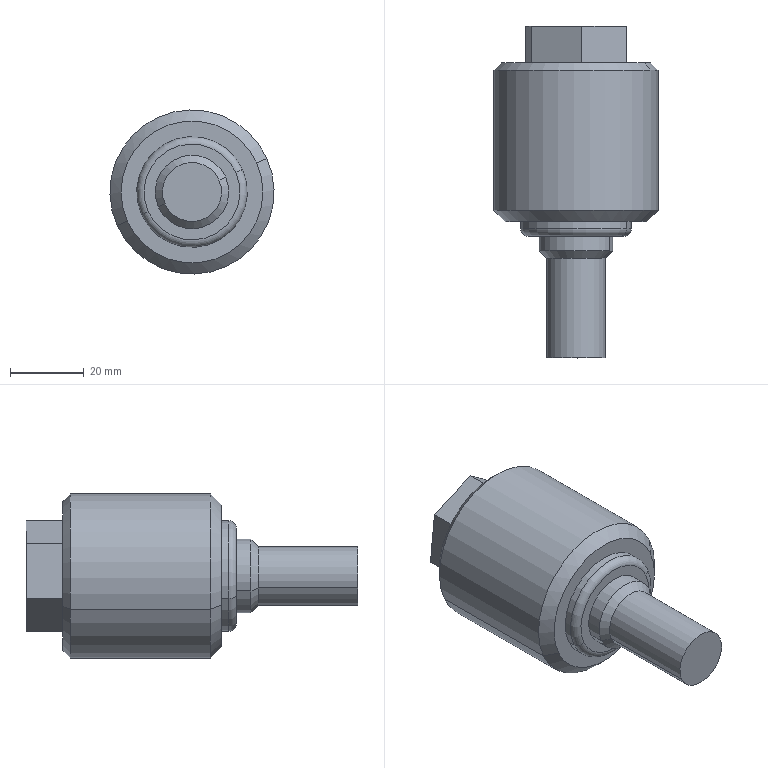Component | SolidWorks | -F-M16150F-1 | 1 solid | 31 faces | box 44.5 x 90 x 44.5 mm | volume 77654 mm3 | plane 11 | cylinder 10 | cone 8 | torus 2 | commonest cylinder face diameters 16 x4 44.5 x2 30 x2 20 x2
STEP:
#1=CARTESIAN_POINT('',(0.8934,52.697,-4.853));
#2=VERTEX_POINT('',#1);
#3=CARTESIAN_POINT('',(1.469,52.697,-4.596));
#4=VERTEX_POINT('',#3);
#5=CARTESIAN_POINT('',(1.181,52.697,-4.724));
#6=DIRECTION('',(-0.,1.,0.));
#7=DIRECTION('',(0.9136,0.,0.4067));
#8=AXIS2_PLACEMENT_3D('',#5,#6,#7);
#9=CIRCLE('',#8,0.315);
#10=EDGE_CURVE('',#2,#4,#9,.T.);
#11=ORIENTED_EDGE('',*,*,#10,.F.);
#12=CARTESIAN_POINT('',(0.8934,53.445,-4.853));
#13=VERTEX_POINT('',#12);
#14=CARTESIAN_POINT('',(0.8934,53.445,-4.853));
#15=DIRECTION('',(-0.,1.,0.));
#16=VECTOR('',#15,39.37);
#17=LINE('',#14,#16);
#18=EDGE_CURVE('',#2,#13,#17,.T.);
#19=ORIENTED_EDGE('',*,*,#18,.T.);
#20=CARTESIAN_POINT('',(1.469,53.445,-4.596));
#21=VERTEX_POINT('',#20);
#22=CARTESIAN_POINT('',(1.181,53.445,-4.724));
#23=DIRECTION('',(-0.,1.,0.));
#24=DIRECTION('',(0.9136,0.,0.4067));
#25=AXIS2_PLACEMENT_3D('',#22,#23,#24);
#26=CIRCLE('',#25,0.315);
#27=EDGE_CURVE('',#13,#21,#26,.T.);
#28=ORIENTED_EDGE('',*,*,#27,.T.);
#29=CARTESIAN_POINT('',(1.469,53.445,-4.596));
#30=DIRECTION('',(-0.,1.,0.));
#31=VECTOR('',#30,39.37);
#32=LINE('',#29,#31);
#33=EDGE_CURVE('',#4,#21,#32,.T.);
#34=ORIENTED_EDGE('',*,*,#33,.F.);
#35=EDGE_LOOP('',(#11,#19,#28,#34));
#36=FACE_OUTER_BOUND('',#35,.T.);
#37=CARTESIAN_POINT('',(1.181,53.445,-4.724));
#38=DIRECTION('',(-0.,1.,0.));
#39=DIRECTION('',(0.9136,0.,0.4067));
#40=AXIS2_PLACEMENT_3D('',#37,#38,#39);
#41=CYLINDRICAL_SURFACE('',#40,0.315);
#42=ADVANCED_FACE('',(#36),#41,.F.);
#43=CARTESIAN_POINT('',(1.181,52.508,-4.724));
#44=VERTEX_POINT('',#43);
#45=CARTESIAN_POINT('',(1.469,52.697,-4.596));
#46=DIRECTION('',(0.7831,0.515,0.3486));
#47=VECTOR('',#46,39.37);
#48=LINE('',#45,#47);
#49=EDGE_CURVE('',#44,#4,#48,.T.);
#50=ORIENTED_EDGE('',*,*,#49,.F.);
#51=CARTESIAN_POINT('',(0.8934,52.697,-4.853));
#52=DIRECTION('',(-0.7831,0.515,-0.3486));
#53=VECTOR('',#52,39.37);
#54=LINE('',#51,#53);
#55=EDGE_CURVE('',#44,#2,#54,.T.);
#56=ORIENTED_EDGE('',*,*,#55,.T.);
#57=ORIENTED_EDGE('',*,*,#10,.T.);
#58=EDGE_LOOP('',(#50,#56,#57));
#59=FACE_OUTER_BOUND('',#58,.T.);
#60=CARTESIAN_POINT('',(1.181,52.697,-4.724));
#61=DIRECTION('',(-0.,1.,0.));
#62=DIRECTION('',(0.9136,0.,0.4067));
#63=AXIS2_PLACEMENT_3D('',#60,#61,#62);
#64=CONICAL_SURFACE('',#63,0.315,1.03);
#65=ADVANCED_FACE('',(#59),#64,.F.);
#66=CARTESIAN_POINT('',(1.909,53.051,-4.4));
#67=VERTEX_POINT('',#66);
#68=CARTESIAN_POINT('',(0.4528,53.051,-5.049));
#69=VERTEX_POINT('',#68);
#70=CARTESIAN_POINT('',(1.181,53.051,-4.724));
#71=DIRECTION('',(-0.,1.,0.));
#72=DIRECTION('',(-0.9136,0.,-0.4067));
#73=AXIS2_PLACEMENT_3D('',#70,#71,#72);
#74=CIRCLE('',#73,0.7972);
#75=EDGE_CURVE('',#67,#69,#74,.T.);
#76=ORIENTED_EDGE('',*,*,#75,.F.);
#77=CARTESIAN_POINT('',(1.981,52.972,-4.368));
#78=VERTEX_POINT('',#77);
#79=CARTESIAN_POINT('',(1.981,52.972,-4.368));
#80=DIRECTION('',(0.646,-0.7071,0.2876));
#81=VECTOR('',#80,39.37);
#82=LINE('',#79,#81);
#83=EDGE_CURVE('',#67,#78,#82,.T.);
#84=ORIENTED_EDGE('',*,*,#83,.T.);
#85=CARTESIAN_POINT('',(0.3808,52.972,-5.081));
#86=VERTEX_POINT('',#85);
#87=CARTESIAN_POINT('',(1.181,52.972,-4.724));
#88=DIRECTION('',(0.,-1.,-0.));
#89=DIRECTION('',(-0.9136,0.,-0.4067));
#90=AXIS2_PLACEMENT_3D('',#87,#88,#89);
#91=CIRCLE('',#90,0.876);
#92=EDGE_CURVE('',#86,#78,#91,.T.);
#93=ORIENTED_EDGE('',*,*,#92,.F.);
#94=CARTESIAN_POINT('',(0.3808,52.972,-5.081));
#95=DIRECTION('',(-0.646,-0.7071,-0.2876));
#96=VECTOR('',#95,39.37);
#97=LINE('',#94,#96);
#98=EDGE_CURVE('',#69,#86,#97,.T.);
#99=ORIENTED_EDGE('',*,*,#98,.F.);
#100=EDGE_LOOP('',(#76,#84,#93,#99));
#101=FACE_OUTER_BOUND('',#100,.T.);
#102=CARTESIAN_POINT('',(1.181,52.972,-4.724));
#103=DIRECTION('',(0.,-1.,-0.));
#104=DIRECTION('',(-0.9136,0.,-0.4067));
#105=AXIS2_PLACEMENT_3D('',#102,#103,#104);
#106=CONICAL_SURFACE('',#105,0.876,0.7854);
#107=ADVANCED_FACE('',(#101),#106,.T.);
#108=CARTESIAN_POINT('',(0.4887,51.358,-5.033));
#109=VERTEX_POINT('',#108);
#110=CARTESIAN_POINT('',(1.873,51.358,-4.416));
#111=VERTEX_POINT('',#110);
#112=CARTESIAN_POINT('',(1.181,51.358,-4.724));
#113=DIRECTION('',(0.,-1.,-0.));
#114=DIRECTION('',(0.9136,0.,0.4067));
#115=AXIS2_PLACEMENT_3D('',#112,#113,#114);
#116=CIRCLE('',#115,0.7579);
#117=EDGE_CURVE('',#109,#111,#116,.T.);
#118=ORIENTED_EDGE('',*,*,#117,.F.);
#119=CARTESIAN_POINT('',(0.3808,51.476,-5.081));
#120=VERTEX_POINT('',#119);
#121=CARTESIAN_POINT('',(0.4887,51.358,-5.033));
#122=DIRECTION('',(-0.646,0.7071,-0.2876));
#123=VECTOR('',#122,39.37);
#124=LINE('',#121,#123);
#125=EDGE_CURVE('',#109,#120,#124,.T.);
#126=ORIENTED_EDGE('',*,*,#125,.T.);
#127=CARTESIAN_POINT('',(1.981,51.476,-4.368));
#128=VERTEX_POINT('',#127);
#129=CARTESIAN_POINT('',(1.181,51.476,-4.724));
#130=DIRECTION('',(-0.,1.,0.));
#131=DIRECTION('',(0.9136,0.,0.4067));
#132=AXIS2_PLACEMENT_3D('',#129,#130,#131);
#133=CIRCLE('',#132,0.876);
#134=EDGE_CURVE('',#128,#120,#133,.T.);
#135=ORIENTED_EDGE('',*,*,#134,.F.);
#136=CARTESIAN_POINT('',(1.873,51.358,-4.416));
#137=DIRECTION('',(0.646,0.7071,0.2876));
#138=VECTOR('',#137,39.37);
#139=LINE('',#136,#138);
#140=EDGE_CURVE('',#111,#128,#139,.T.);
#141=ORIENTED_EDGE('',*,*,#140,.F.);
#142=EDGE_LOOP('',(#118,#126,#135,#141));
#143=FACE_OUTER_BOUND('',#142,.T.);
#144=CARTESIAN_POINT('',(1.181,51.358,-4.724));
#145=DIRECTION('',(-0.,1.,0.));
#146=DIRECTION('',(0.9136,0.,0.4067));
#147=AXIS2_PLACEMENT_3D('',#144,#145,#146);
#148=CONICAL_SURFACE('',#147,0.7579,0.7854);
#149=ADVANCED_FACE('',(#143),#148,.T.);
#150=CARTESIAN_POINT('',(0.7135,51.201,-4.933));
#151=VERTEX_POINT('',#150);
#152=CARTESIAN_POINT('',(1.649,51.201,-4.516));
#153=VERTEX_POINT('',#152);
#154=CARTESIAN_POINT('',(1.181,51.201,-4.724));
#155=DIRECTION('',(0.,-1.,-0.));
#156=DIRECTION('',(0.9136,0.,0.4067));
#157=AXIS2_PLACEMENT_3D('',#154,#155,#156);
#158=CIRCLE('',#157,0.5118);
#159=EDGE_CURVE('',#151,#153,#158,.T.);
#160=ORIENTED_EDGE('',*,*,#159,.F.);
#161=CARTESIAN_POINT('',(0.6416,51.28,-4.965));
#162=VERTEX_POINT('',#161);
#163=CARTESIAN_POINT('',(0.7135,51.28,-4.933));
#164=DIRECTION('',(0.4067,0.,-0.9136));
#165=DIRECTION('',(-0.9136,0.,-0.4067));
#166=AXIS2_PLACEMENT_3D('',#163,#164,#165);
#167=CIRCLE('',#166,0.07874);
#168=EDGE_CURVE('',#151,#162,#167,.T.);
#169=ORIENTED_EDGE('',*,*,#168,.T.);
#170=CARTESIAN_POINT('',(1.721,51.28,-4.484));
#171=VERTEX_POINT('',#170);
#172=CARTESIAN_POINT('',(1.181,51.28,-4.724));
#173=DIRECTION('',(-0.,1.,0.));
#174=DIRECTION('',(0.9136,0.,0.4067));
#175=AXIS2_PLACEMENT_3D('',#172,#173,#174);
#176=CIRCLE('',#175,0.5906);
#177=EDGE_CURVE('',#171,#162,#176,.T.);
#178=ORIENTED_EDGE('',*,*,#177,.F.);
#179=CARTESIAN_POINT('',(1.649,51.28,-4.516));
#180=DIRECTION('',(-0.4067,-0.,0.9136));
#181=DIRECTION('',(0.9136,0.,0.4067));
#182=AXIS2_PLACEMENT_3D('',#179,#180,#181);
#183=CIRCLE('',#182,0.07874);
#184=EDGE_CURVE('',#153,#171,#183,.T.);
#185=ORIENTED_EDGE('',*,*,#184,.F.);
#186=EDGE_LOOP('',(#160,#169,#178,#185));
#187=FACE_OUTER_BOUND('',#186,.T.);
#188=CARTESIAN_POINT('',(1.181,51.28,-4.724));
#189=DIRECTION('',(-0.,1.,0.));
#190=DIRECTION('',(0.9136,-0.,0.4067));
#191=AXIS2_PLACEMENT_3D('',#188,#189,#190);
#192=TOROIDAL_SURFACE('',#191,0.5118,0.07874);
#193=ADVANCED_FACE('',(#187),#192,.T.);
#194=CARTESIAN_POINT('',(0.8934,50.965,-4.853));
#195=VERTEX_POINT('',#194);
#196=CARTESIAN_POINT('',(1.469,50.965,-4.596));
#197=VERTEX_POINT('',#196);
#198=CARTESIAN_POINT('',(1.181,50.965,-4.724));
#199=DIRECTION('',(0.,-1.,-0.));
#200=DIRECTION('',(-0.9136,0.,-0.4067));
#201=AXIS2_PLACEMENT_3D('',#198,#199,#200);
#202=CIRCLE('',#201,0.315);
#203=EDGE_CURVE('',#195,#197,#202,.T.);
#204=ORIENTED_EDGE('',*,*,#203,.F.);
#205=CARTESIAN_POINT('',(0.8214,51.043,-4.885));
#206=VERTEX_POINT('',#205);
#207=CARTESIAN_POINT('',(0.8934,50.965,-4.853));
#208=DIRECTION('',(-0.646,0.7071,-0.2876));
#209=VECTOR('',#208,39.37);
#210=LINE('',#207,#209);
#211=EDGE_CURVE('',#195,#206,#210,.T.);
#212=ORIENTED_EDGE('',*,*,#211,.T.);
#213=CARTESIAN_POINT('',(1.541,51.043,-4.564));
#214=VERTEX_POINT('',#213);
#215=CARTESIAN_POINT('',(1.181,51.043,-4.724));
#216=DIRECTION('',(-0.,1.,0.));
#217=DIRECTION('',(0.9136,0.,0.4067));
#218=AXIS2_PLACEMENT_3D('',#215,#216,#217);
#219=CIRCLE('',#218,0.3937);
#220=EDGE_CURVE('',#214,#206,#219,.T.);
#221=ORIENTED_EDGE('',*,*,#220,.F.);
#222=CARTESIAN_POINT('',(1.469,50.965,-4.596));
#223=DIRECTION('',(0.646,0.7071,0.2876));
#224=VECTOR('',#223,39.37);
#225=LINE('',#222,#224);
#226=EDGE_CURVE('',#197,#214,#225,.T.);
#227=ORIENTED_EDGE('',*,*,#226,.F.);
#228=EDGE_LOOP('',(#204,#212,#221,#227));
#229=FACE_OUTER_BOUND('',#228,.T.);
#230=CARTESIAN_POINT('',(1.181,50.965,-4.724));
#231=DIRECTION('',(-0.,1.,0.));
#232=DIRECTION('',(0.9136,0.,0.4067));
#233=AXIS2_PLACEMENT_3D('',#230,#231,#232);
#234=CONICAL_SURFACE('',#233,0.315,0.7854);
#235=ADVANCED_FACE('',(#229),#234,.T.);
#236=ORIENTED_EDGE('',*,*,#92,.T.);
#237=CARTESIAN_POINT('',(1.981,38.509,-4.368));
#238=DIRECTION('',(0.,-1.,-0.));
#239=VECTOR('',#238,39.37);
#240=LINE('',#237,#239);
#241=EDGE_CURVE('',#78,#128,#240,.T.);
#242=ORIENTED_EDGE('',*,*,#241,.T.);
#243=ORIENTED_EDGE('',*,*,#134,.T.);
#244=CARTESIAN_POINT('',(0.3808,38.509,-5.081));
#245=DIRECTION('',(0.,-1.,-0.));
#246=VECTOR('',#245,39.37);
#247=LINE('',#244,#246);
#248=EDGE_CURVE('',#86,#120,#247,.T.);
#249=ORIENTED_EDGE('',*,*,#248,.F.);
#250=EDGE_LOOP('',(#236,#242,#243,#249));
#251=FACE_OUTER_BOUND('',#250,.T.);
#252=CARTESIAN_POINT('',(1.181,38.509,-4.724));
#253=DIRECTION('',(0.,-1.,-0.));
#254=DIRECTION('',(-0.9136,0.,-0.4067));
#255=AXIS2_PLACEMENT_3D('',#252,#253,#254);
#256=CYLINDRICAL_SURFACE('',#255,0.876);
#257=ADVANCED_FACE('',(#251),#256,.T.);
#258=CARTESIAN_POINT('',(0.6416,51.358,-4.965));
#259=VERTEX_POINT('',#258);
#260=CARTESIAN_POINT('',(1.721,51.358,-4.484));
#261=VERTEX_POINT('',#260);
#262=CARTESIAN_POINT('',(1.181,51.358,-4.724));
#263=DIRECTION('',(0.,-1.,-0.));
#264=DIRECTION('',(-0.9136,0.,-0.4067));
#265=AXIS2_PLACEMENT_3D('',#262,#263,#264);
#266=CIRCLE('',#265,0.5906);
#267=EDGE_CURVE('',#259,#261,#266,.T.);
#268=ORIENTED_EDGE('',*,*,#267,.T.);
#269=CARTESIAN_POINT('',(1.721,38.509,-4.484));
#270=DIRECTION('',(0.,-1.,-0.));
#271=VECTOR('',#270,39.37);
#272=LINE('',#269,#271);
#273=EDGE_CURVE('',#261,#171,#272,.T.);
#274=ORIENTED_EDGE('',*,*,#273,.T.);
#275=ORIENTED_EDGE('',*,*,#177,.T.);
#276=CARTESIAN_POINT('',(0.6416,38.509,-4.965));
#277=DIRECTION('',(0.,-1.,-0.));
#278=VECTOR('',#277,39.37);
#279=LINE('',#276,#278);
#280=EDGE_CURVE('',#259,#162,#279,.T.);
#281=ORIENTED_EDGE('',*,*,#280,.F.);
#282=EDGE_LOOP('',(#268,#274,#275,#281));
#283=FACE_OUTER_BOUND('',#282,.T.);
#284=CARTESIAN_POINT('',(1.181,38.509,-4.724));
#285=DIRECTION('',(0.,-1.,-0.));
#286=DIRECTION('',(-0.9136,0.,-0.4067));
#287=AXIS2_PLACEMENT_3D('',#284,#285,#286);
#288=CYLINDRICAL_SURFACE('',#287,0.5906);
#289=ADVANCED_FACE('',(#283),#288,.T.);
#290=CARTESIAN_POINT('',(0.8214,51.201,-4.885));
#291=VERTEX_POINT('',#290);
#292=CARTESIAN_POINT('',(1.541,51.201,-4.564));
#293=VERTEX_POINT('',#292);
#294=CARTESIAN_POINT('',(1.181,51.201,-4.724));
#295=DIRECTION('',(0.,-1.,-0.));
#296=DIRECTION('',(-0.9136,0.,-0.4067));
#297=AXIS2_PLACEMENT_3D('',#294,#295,#296);
#298=CIRCLE('',#297,0.3937);
#299=EDGE_CURVE('',#291,#293,#298,.T.);
#300=ORIENTED_EDGE('',*,*,#299,.T.);
#301=CARTESIAN_POINT('',(1.541,38.509,-4.564));
#302=DIRECTION('',(0.,-1.,-0.));
#303=VECTOR('',#302,39.37);
#304=LINE('',#301,#303);
#305=EDGE_CURVE('',#293,#214,#304,.T.);
#306=ORIENTED_EDGE('',*,*,#305,.T.);
#307=ORIENTED_EDGE('',*,*,#220,.T.);
#308=CARTESIAN_POINT('',(0.8214,38.509,-4.885));
#309=DIRECTION('',(0.,-1.,-0.));
#310=VECTOR('',#309,39.37);
#311=LINE('',#308,#310);
#312=EDGE_CURVE('',#291,#206,#311,.T.);
#313=ORIENTED_EDGE('',*,*,#312,.F.);
#314=EDGE_LOOP('',(#300,#306,#307,#313));
#315=FACE_OUTER_BOUND('',#314,.T.);
#316=CARTESIAN_POINT('',(1.181,38.509,-4.724));
#317=DIRECTION('',(0.,-1.,-0.));
#318=DIRECTION('',(-0.9136,0.,-0.4067));
#319=AXIS2_PLACEMENT_3D('',#316,#317,#318);
#320=CYLINDRICAL_SURFACE('',#319,0.3937);
#321=ADVANCED_FACE('',(#315),#320,.T.);
#322=ORIENTED_EDGE('',*,*,#203,.T.);
#323=CARTESIAN_POINT('',(1.469,49.902,-4.596));
#324=VERTEX_POINT('',#323);
#325=CARTESIAN_POINT('',(1.469,38.509,-4.596));
#326=DIRECTION('',(0.,-1.,-0.));
#327=VECTOR('',#326,39.37);
#328=LINE('',#325,#327);
#329=EDGE_CURVE('',#197,#324,#328,.T.);
#330=ORIENTED_EDGE('',*,*,#329,.T.);
#331=CARTESIAN_POINT('',(0.8934,49.902,-4.853));
#332=VERTEX_POINT('',#331);
#333=CARTESIAN_POINT('',(1.181,49.902,-4.724));
#334=DIRECTION('',(0.,-1.,-0.));
#335=DIRECTION('',(-0.9136,0.,-0.4067));
#336=AXIS2_PLACEMENT_3D('',#333,#334,#335);
#337=CIRCLE('',#336,0.315);
#338=EDGE_CURVE('',#332,#324,#337,.T.);
#339=ORIENTED_EDGE('',*,*,#338,.F.);
#340=CARTESIAN_POINT('',(0.8934,38.509,-4.853));
#341=DIRECTION('',(0.,-1.,-0.));
#342=VECTOR('',#341,39.37);
#343=LINE('',#340,#342);
#344=EDGE_CURVE('',#195,#332,#343,.T.);
#345=ORIENTED_EDGE('',*,*,#344,.F.);
#346=EDGE_LOOP('',(#322,#330,#339,#345));
#347=FACE_OUTER_BOUND('',#346,.T.);
#348=CARTESIAN_POINT('',(1.181,38.509,-4.724));
#349=DIRECTION('',(0.,-1.,-0.));
#350=DIRECTION('',(-0.9136,0.,-0.4067));
#351=AXIS2_PLACEMENT_3D('',#348,#349,#350);
#352=CYLINDRICAL_SURFACE('',#351,0.315);
#353=ADVANCED_FACE('',(#347),#352,.T.);
#354=ORIENTED_EDGE('',*,*,#338,.T.);
#355=CARTESIAN_POINT('',(1.181,49.902,-4.724));
#356=DIRECTION('',(0.,-1.,-0.));
#357=DIRECTION('',(-0.9136,0.,-0.4067));
#358=AXIS2_PLACEMENT_3D('',#355,#356,#357);
#359=CIRCLE('',#358,0.315);
#360=EDGE_CURVE('',#324,#332,#359,.T.);
#361=ORIENTED_EDGE('',*,*,#360,.T.);
#362=EDGE_LOOP('',(#354,#361));
#363=FACE_OUTER_BOUND('',#362,.T.);
#364=CARTESIAN_POINT('',(1.181,49.902,-4.724));
#365=DIRECTION('',(-0.,1.,0.));
#366=DIRECTION('',(0.9136,-0.,0.4067));
#367=AXIS2_PLACEMENT_3D('',#364,#365,#366);
#368=PLANE('',#367);
#369=ADVANCED_FACE('',(#363),#368,.F.);
#370=ORIENTED_EDGE('',*,*,#329,.F.);
#371=CARTESIAN_POINT('',(1.181,50.965,-4.724));
#372=DIRECTION('',(0.,-1.,-0.));
#373=DIRECTION('',(-0.9136,0.,-0.4067));
#374=AXIS2_PLACEMENT_3D('',#371,#372,#373);
#375=CIRCLE('',#374,0.315);
#376=EDGE_CURVE('',#197,#195,#375,.T.);
#377=ORIENTED_EDGE('',*,*,#376,.T.);
#378=ORIENTED_EDGE('',*,*,#344,.T.);
#379=ORIENTED_EDGE('',*,*,#360,.F.);
#380=EDGE_LOOP('',(#370,#377,#378,#379));
#381=FACE_OUTER_BOUND('',#380,.T.);
#382=CARTESIAN_POINT('',(1.181,38.509,-4.724));
#383=DIRECTION('',(0.,-1.,-0.));
#384=DIRECTION('',(-0.9136,0.,-0.4067));
#385=AXIS2_PLACEMENT_3D('',#382,#383,#384);
#386=CYLINDRICAL_SURFACE('',#385,0.315);
#387=ADVANCED_FACE('',(#381),#386,.T.);
#388=ORIENTED_EDGE('',*,*,#305,.F.);
#389=CARTESIAN_POINT('',(1.181,51.201,-4.724));
#390=DIRECTION('',(0.,-1.,-0.));
#391=DIRECTION('',(-0.9136,0.,-0.4067));
#392=AXIS2_PLACEMENT_3D('',#389,#390,#391);
#393=CIRCLE('',#392,0.3937);
#394=EDGE_CURVE('',#293,#291,#393,.T.);
#395=ORIENTED_EDGE('',*,*,#394,.T.);
#396=ORIENTED_EDGE('',*,*,#312,.T.);
#397=CARTESIAN_POINT('',(1.181,51.043,-4.724));
#398=DIRECTION('',(-0.,1.,0.));
#399=DIRECTION('',(0.9136,0.,0.4067));
#400=AXIS2_PLACEMENT_3D('',#397,#398,#399);
#401=CIRCLE('',#400,0.3937);
#402=EDGE_CURVE('',#206,#214,#401,.T.);
#403=ORIENTED_EDGE('',*,*,#402,.T.);
#404=EDGE_LOOP('',(#388,#395,#396,#403));
#405=FACE_OUTER_BOUND('',#404,.T.);
#406=CARTESIAN_POINT('',(1.181,38.509,-4.724));
#407=DIRECTION('',(0.,-1.,-0.));
#408=DIRECTION('',(-0.9136,0.,-0.4067));
#409=AXIS2_PLACEMENT_3D('',#406,#407,#408);
#410=CYLINDRICAL_SURFACE('',#409,0.3937);
#411=ADVANCED_FACE('',(#405),#410,.T.);
#412=CARTESIAN_POINT('',(1.181,51.201,-4.724));
#413=DIRECTION('',(0.,-1.,-0.));
#414=DIRECTION('',(0.9136,0.,0.4067));
#415=AXIS2_PLACEMENT_3D('',#412,#413,#414);
#416=CIRCLE('',#415,0.5118);
#417=EDGE_CURVE('',#153,#151,#416,.T.);
#418=ORIENTED_EDGE('',*,*,#417,.T.);
#419=ORIENTED_EDGE('',*,*,#159,.T.);
#420=EDGE_LOOP('',(#418,#419));
#421=FACE_OUTER_BOUND('',#420,.T.);
#422=ORIENTED_EDGE('',*,*,#299,.F.);
#423=ORIENTED_EDGE('',*,*,#394,.F.);
#424=EDGE_LOOP('',(#422,#423));
#425=FACE_BOUND('',#424,.T.);
#426=CARTESIAN_POINT('',(1.341,51.201,-5.084));
#427=DIRECTION('',(-0.,1.,0.));
#428=DIRECTION('',(0.9136,-0.,0.4067));
#429=AXIS2_PLACEMENT_3D('',#426,#427,#428);
#430=PLANE('',#429);
#431=ADVANCED_FACE('',(#421,#425),#430,.F.);
#432=ORIENTED_EDGE('',*,*,#273,.F.);
#433=CARTESIAN_POINT('',(1.181,51.358,-4.724));
#434=DIRECTION('',(0.,-1.,-0.));
#435=DIRECTION('',(-0.9136,0.,-0.4067));
#436=AXIS2_PLACEMENT_3D('',#433,#434,#435);
#437=CIRCLE('',#436,0.5906);
#438=EDGE_CURVE('',#261,#259,#437,.T.);
#439=ORIENTED_EDGE('',*,*,#438,.T.);
#440=ORIENTED_EDGE('',*,*,#280,.T.);
#441=CARTESIAN_POINT('',(1.181,51.28,-4.724));
#442=DIRECTION('',(-0.,1.,0.));
#443=DIRECTION('',(0.9136,0.,0.4067));
#444=AXIS2_PLACEMENT_3D('',#441,#442,#443);
#445=CIRCLE('',#444,0.5906);
#446=EDGE_CURVE('',#162,#171,#445,.T.);
#447=ORIENTED_EDGE('',*,*,#446,.T.);
#448=EDGE_LOOP('',(#432,#439,#440,#447));
#449=FACE_OUTER_BOUND('',#448,.T.);
#450=CARTESIAN_POINT('',(1.181,38.509,-4.724));
#451=DIRECTION('',(0.,-1.,-0.));
#452=DIRECTION('',(-0.9136,0.,-0.4067));
#453=AXIS2_PLACEMENT_3D('',#450,#451,#452);
#454=CYLINDRICAL_SURFACE('',#453,0.5906);
#455=ADVANCED_FACE('',(#449),#454,.T.);
#456=CARTESIAN_POINT('',(1.181,51.358,-4.724));
#457=DIRECTION('',(0.,-1.,-0.));
#458=DIRECTION('',(0.9136,0.,0.4067));
#459=AXIS2_PLACEMENT_3D('',#456,#457,#458);
#460=CIRCLE('',#459,0.7579);
#461=EDGE_CURVE('',#111,#109,#460,.T.);
#462=ORIENTED_EDGE('',*,*,#461,.T.);
#463=ORIENTED_EDGE('',*,*,#117,.T.);
#464=EDGE_LOOP('',(#462,#463));
#465=FACE_OUTER_BOUND('',#464,.T.);
#466=ORIENTED_EDGE('',*,*,#267,.F.);
#467=ORIENTED_EDGE('',*,*,#438,.F.);
#468=EDGE_LOOP('',(#466,#467));
#469=FACE_BOUND('',#468,.T.);
#470=CARTESIAN_POINT('',(1.421,51.358,-5.264));
#471=DIRECTION('',(-0.,1.,0.));
#472=DIRECTION('',(0.9136,-0.,0.4067));
#473=AXIS2_PLACEMENT_3D('',#470,#471,#472);
#474=PLANE('',#473);
#475=ADVANCED_FACE('',(#465,#469),#474,.F.);
#476=ORIENTED_EDGE('',*,*,#241,.F.);
#477=CARTESIAN_POINT('',(1.181,52.972,-4.724));
#478=DIRECTION('',(0.,-1.,-0.));
#479=DIRECTION('',(-0.9136,0.,-0.4067));
#480=AXIS2_PLACEMENT_3D('',#477,#478,#479);
#481=CIRCLE('',#480,0.876);
#482=EDGE_CURVE('',#78,#86,#481,.T.);
#483=ORIENTED_EDGE('',*,*,#482,.T.);
#484=ORIENTED_EDGE('',*,*,#248,.T.);
#485=CARTESIAN_POINT('',(1.181,51.476,-4.724));
#486=DIRECTION('',(-0.,1.,0.));
#487=DIRECTION('',(0.9136,0.,0.4067));
#488=AXIS2_PLACEMENT_3D('',#485,#486,#487);
#489=CIRCLE('',#488,0.876);
#490=EDGE_CURVE('',#120,#128,#489,.T.);
#491=ORIENTED_EDGE('',*,*,#490,.T.);
#492=EDGE_LOOP('',(#476,#483,#484,#491));
#493=FACE_OUTER_BOUND('',#492,.T.);
#494=CARTESIAN_POINT('',(1.181,38.509,-4.724));
#495=DIRECTION('',(0.,-1.,-0.));
#496=DIRECTION('',(-0.9136,0.,-0.4067));
#497=AXIS2_PLACEMENT_3D('',#494,#495,#496);
#498=CYLINDRICAL_SURFACE('',#497,0.876);
#499=ADVANCED_FACE('',(#493),#498,.T.);
#500=CARTESIAN_POINT('',(1.181,53.051,-4.724));
#501=DIRECTION('',(-0.,1.,0.));
#502=DIRECTION('',(-0.9136,0.,-0.4067));
#503=AXIS2_PLACEMENT_3D('',#500,#501,#502);
#504=CIRCLE('',#503,0.7972);
#505=EDGE_CURVE('',#69,#67,#504,.T.);
#506=ORIENTED_EDGE('',*,*,#505,.T.);
#507=ORIENTED_EDGE('',*,*,#75,.T.);
#508=EDGE_LOOP('',(#506,#507));
#509=FACE_OUTER_BOUND('',#508,.T.);
#510=CARTESIAN_POINT('',(1.721,53.051,-4.484));
#511=VERTEX_POINT('',#510);
#512=CARTESIAN_POINT('',(1.243,53.051,-4.137));
#513=VERTEX_POINT('',#512);
#514=CARTESIAN_POINT('',(1.243,53.051,-4.137));
#515=DIRECTION('',(-0.809,-0.,0.5878));
#516=VECTOR('',#515,39.37);
#517=LINE('',#514,#516);
#518=EDGE_CURVE('',#511,#513,#517,.T.);
#519=ORIENTED_EDGE('',*,*,#518,.T.);
#520=CARTESIAN_POINT('',(0.7033,53.051,-4.377));
#521=VERTEX_POINT('',#520);
#522=CARTESIAN_POINT('',(0.7033,53.051,-4.377));
#523=DIRECTION('',(-0.9136,0.,-0.4067));
#524=VECTOR('',#523,39.37);
#525=LINE('',#522,#524);
#526=EDGE_CURVE('',#513,#521,#525,.T.);
#527=ORIENTED_EDGE('',*,*,#526,.T.);
#528=CARTESIAN_POINT('',(0.6416,53.051,-4.965));
#529=VERTEX_POINT('',#528);
#530=CARTESIAN_POINT('',(0.6416,53.051,-4.965));
#531=DIRECTION('',(-0.1046,0.,-0.9945));
#532=VECTOR('',#531,39.37);
#533=LINE('',#530,#532);
#534=EDGE_CURVE('',#521,#529,#533,.T.);
#535=ORIENTED_EDGE('',*,*,#534,.T.);
#536=CARTESIAN_POINT('',(1.119,53.051,-5.312));
#537=VERTEX_POINT('',#536);
#538=CARTESIAN_POINT('',(1.119,53.051,-5.312));
#539=DIRECTION('',(0.809,0.,-0.5878));
#540=VECTOR('',#539,39.37);
#541=LINE('',#538,#540);
#542=EDGE_CURVE('',#529,#537,#541,.T.);
#543=ORIENTED_EDGE('',*,*,#542,.T.);
#544=CARTESIAN_POINT('',(1.659,53.051,-5.072));
#545=VERTEX_POINT('',#544);
#546=CARTESIAN_POINT('',(1.659,53.051,-5.072));
#547=DIRECTION('',(0.9136,-0.,0.4067));
#548=VECTOR('',#547,39.37);
#549=LINE('',#546,#548);
#550=EDGE_CURVE('',#537,#545,#549,.T.);
#551=ORIENTED_EDGE('',*,*,#550,.T.);
#552=CARTESIAN_POINT('',(1.721,53.051,-4.484));
#553=DIRECTION('',(0.1046,-0.,0.9945));
#554=VECTOR('',#553,39.37);
#555=LINE('',#552,#554);
#556=EDGE_CURVE('',#545,#511,#555,.T.);
#557=ORIENTED_EDGE('',*,*,#556,.T.);
#558=EDGE_LOOP('',(#519,#527,#535,#543,#551,#557));
#559=FACE_BOUND('',#558,.T.);
#560=CARTESIAN_POINT('',(1.537,53.051,-5.525));
#561=DIRECTION('',(0.,-1.,-0.));
#562=DIRECTION('',(-0.9136,0.,-0.4067));
#563=AXIS2_PLACEMENT_3D('',#560,#561,#562);
#564=PLANE('',#563);
#565=ADVANCED_FACE('',(#509,#559),#564,.F.);
#566=CARTESIAN_POINT('',(1.181,53.445,-4.724));
#567=DIRECTION('',(-0.,1.,0.));
#568=DIRECTION('',(0.9136,0.,0.4067));
#569=AXIS2_PLACEMENT_3D('',#566,#567,#568);
#570=CIRCLE('',#569,0.315);
#571=EDGE_CURVE('',#21,#13,#570,.T.);
#572=ORIENTED_EDGE('',*,*,#571,.F.);
#573=ORIENTED_EDGE('',*,*,#27,.F.);
#574=EDGE_LOOP('',(#572,#573));
#575=FACE_BOUND('',#574,.T.);
#576=CARTESIAN_POINT('',(1.721,53.445,-4.484));
#577=VERTEX_POINT('',#576);
#578=CARTESIAN_POINT('',(1.243,53.445,-4.137));
#579=VERTEX_POINT('',#578);
#580=CARTESIAN_POINT('',(1.243,53.445,-4.137));
#581=DIRECTION('',(-0.809,-0.,0.5878));
#582=VECTOR('',#581,39.37);
#583=LINE('',#580,#582);
#584=EDGE_CURVE('',#577,#579,#583,.T.);
#585=ORIENTED_EDGE('',*,*,#584,.F.);
#586=CARTESIAN_POINT('',(1.659,53.445,-5.072));
#587=VERTEX_POINT('',#586);
#588=CARTESIAN_POINT('',(1.721,53.445,-4.484));
#589=DIRECTION('',(0.1046,-0.,0.9945));
#590=VECTOR('',#589,39.37);
#591=LINE('',#588,#590);
#592=EDGE_CURVE('',#587,#577,#591,.T.);
#593=ORIENTED_EDGE('',*,*,#592,.F.);
#594=CARTESIAN_POINT('',(1.119,53.445,-5.312));
#595=VERTEX_POINT('',#594);
#596=CARTESIAN_POINT('',(1.659,53.445,-5.072));
#597=DIRECTION('',(0.9136,-0.,0.4067));
#598=VECTOR('',#597,39.37);
#599=LINE('',#596,#598);
#600=EDGE_CURVE('',#595,#587,#599,.T.);
#601=ORIENTED_EDGE('',*,*,#600,.F.);
#602=CARTESIAN_POINT('',(0.6416,53.445,-4.965));
#603=VERTEX_POINT('',#602);
#604=CARTESIAN_POINT('',(1.119,53.445,-5.312));
#605=DIRECTION('',(0.809,0.,-0.5878));
#606=VECTOR('',#605,39.37);
#607=LINE('',#604,#606);
#608=EDGE_CURVE('',#603,#595,#607,.T.);
#609=ORIENTED_EDGE('',*,*,#608,.F.);
#610=CARTESIAN_POINT('',(0.7033,53.445,-4.377));
#611=VERTEX_POINT('',#610);
#612=CARTESIAN_POINT('',(0.6416,53.445,-4.965));
#613=DIRECTION('',(-0.1046,0.,-0.9945));
#614=VECTOR('',#613,39.37);
#615=LINE('',#612,#614);
#616=EDGE_CURVE('',#611,#603,#615,.T.);
#617=ORIENTED_EDGE('',*,*,#616,.F.);
#618=CARTESIAN_POINT('',(0.7033,53.445,-4.377));
#619=DIRECTION('',(-0.9136,0.,-0.4067));
#620=VECTOR('',#619,39.37);
#621=LINE('',#618,#620);
#622=EDGE_CURVE('',#579,#611,#621,.T.);
#623=ORIENTED_EDGE('',*,*,#622,.F.);
#624=EDGE_LOOP('',(#585,#593,#601,#609,#617,#623));
#625=FACE_OUTER_BOUND('',#624,.T.);
#626=CARTESIAN_POINT('',(1.421,53.445,-5.264));
#627=DIRECTION('',(0.,-1.,-0.));
#628=DIRECTION('',(-0.9136,0.,-0.4067));
#629=AXIS2_PLACEMENT_3D('',#626,#627,#628);
#630=PLANE('',#629);
#631=ADVANCED_FACE('',(#575,#625),#630,.F.);
#632=ORIENTED_EDGE('',*,*,#211,.F.);
#633=ORIENTED_EDGE('',*,*,#376,.F.);
#634=ORIENTED_EDGE('',*,*,#226,.T.);
#635=ORIENTED_EDGE('',*,*,#402,.F.);
#636=EDGE_LOOP('',(#632,#633,#634,#635));
#637=FACE_OUTER_BOUND('',#636,.T.);
#638=CARTESIAN_POINT('',(1.181,50.965,-4.724));
#639=DIRECTION('',(-0.,1.,0.));
#640=DIRECTION('',(0.9136,0.,0.4067));
#641=AXIS2_PLACEMENT_3D('',#638,#639,#640);
#642=CONICAL_SURFACE('',#641,0.315,0.7854);
#643=ADVANCED_FACE('',(#637),#642,.T.);
#644=ORIENTED_EDGE('',*,*,#168,.F.);
#645=ORIENTED_EDGE('',*,*,#417,.F.);
#646=ORIENTED_EDGE('',*,*,#184,.T.);
#647=ORIENTED_EDGE('',*,*,#446,.F.);
#648=EDGE_LOOP('',(#644,#645,#646,#647));
#649=FACE_OUTER_BOUND('',#648,.T.);
#650=CARTESIAN_POINT('',(1.181,51.28,-4.724));
#651=DIRECTION('',(-0.,1.,0.));
#652=DIRECTION('',(0.9136,-0.,0.4067));
#653=AXIS2_PLACEMENT_3D('',#650,#651,#652);
#654=TOROIDAL_SURFACE('',#653,0.5118,0.07874);
#655=ADVANCED_FACE('',(#649),#654,.T.);
#656=ORIENTED_EDGE('',*,*,#125,.F.);
#657=ORIENTED_EDGE('',*,*,#461,.F.);
#658=ORIENTED_EDGE('',*,*,#140,.T.);
#659=ORIENTED_EDGE('',*,*,#490,.F.);
#660=EDGE_LOOP('',(#656,#657,#658,#659));
#661=FACE_OUTER_BOUND('',#660,.T.);
#662=CARTESIAN_POINT('',(1.181,51.358,-4.724));
#663=DIRECTION('',(-0.,1.,0.));
#664=DIRECTION('',(0.9136,0.,0.4067));
#665=AXIS2_PLACEMENT_3D('',#662,#663,#664);
#666=CONICAL_SURFACE('',#665,0.7579,0.7854);
#667=ADVANCED_FACE('',(#661),#666,.T.);
#668=ORIENTED_EDGE('',*,*,#83,.F.);
#669=ORIENTED_EDGE('',*,*,#505,.F.);
#670=ORIENTED_EDGE('',*,*,#98,.T.);
#671=ORIENTED_EDGE('',*,*,#482,.F.);
#672=EDGE_LOOP('',(#668,#669,#670,#671));
#673=FACE_OUTER_BOUND('',#672,.T.);
#674=CARTESIAN_POINT('',(1.181,52.972,-4.724));
#675=DIRECTION('',(0.,-1.,-0.));
#676=DIRECTION('',(-0.9136,0.,-0.4067));
#677=AXIS2_PLACEMENT_3D('',#674,#675,#676);
#678=CONICAL_SURFACE('',#677,0.876,0.7854);
#679=ADVANCED_FACE('',(#673),#678,.T.);
#680=ORIENTED_EDGE('',*,*,#584,.T.);
#681=CARTESIAN_POINT('',(1.243,53.051,-4.137));
#682=DIRECTION('',(-0.,1.,0.));
#683=VECTOR('',#682,39.37);
#684=LINE('',#681,#683);
#685=EDGE_CURVE('',#513,#579,#684,.T.);
#686=ORIENTED_EDGE('',*,*,#685,.F.);
#687=ORIENTED_EDGE('',*,*,#518,.F.);
#688=CARTESIAN_POINT('',(1.721,53.051,-4.484));
#689=DIRECTION('',(-0.,1.,0.));
#690=VECTOR('',#689,39.37);
#691=LINE('',#688,#690);
#692=EDGE_CURVE('',#511,#577,#691,.T.);
#693=ORIENTED_EDGE('',*,*,#692,.T.);
#694=EDGE_LOOP('',(#680,#686,#687,#693));
#695=FACE_OUTER_BOUND('',#694,.T.);
#696=CARTESIAN_POINT('',(1.243,53.051,-4.137));
#697=DIRECTION('',(-0.5878,0.,-0.809));
#698=DIRECTION('',(-0.809,-0.,0.5878));
#699=AXIS2_PLACEMENT_3D('',#696,#697,#698);
#700=PLANE('',#699);
#701=ADVANCED_FACE('',(#695),#700,.F.);
#702=ORIENTED_EDGE('',*,*,#622,.T.);
#703=CARTESIAN_POINT('',(0.7033,53.051,-4.377));
#704=DIRECTION('',(-0.,1.,0.));
#705=VECTOR('',#704,39.37);
#706=LINE('',#703,#705);
#707=EDGE_CURVE('',#521,#611,#706,.T.);
#708=ORIENTED_EDGE('',*,*,#707,.F.);
#709=ORIENTED_EDGE('',*,*,#526,.F.);
#710=ORIENTED_EDGE('',*,*,#685,.T.);
#711=EDGE_LOOP('',(#702,#708,#709,#710));
#712=FACE_OUTER_BOUND('',#711,.T.);
#713=CARTESIAN_POINT('',(0.7033,53.051,-4.377));
#714=DIRECTION('',(0.4067,0.,-0.9136));
#715=DIRECTION('',(-0.9136,0.,-0.4067));
#716=AXIS2_PLACEMENT_3D('',#713,#714,#715);
#717=PLANE('',#716);
#718=ADVANCED_FACE('',(#712),#717,.F.);
#719=ORIENTED_EDGE('',*,*,#616,.T.);
#720=CARTESIAN_POINT('',(0.6416,53.051,-4.965));
#721=DIRECTION('',(-0.,1.,0.));
#722=VECTOR('',#721,39.37);
#723=LINE('',#720,#722);
#724=EDGE_CURVE('',#529,#603,#723,.T.);
#725=ORIENTED_EDGE('',*,*,#724,.F.);
#726=ORIENTED_EDGE('',*,*,#534,.F.);
#727=ORIENTED_EDGE('',*,*,#707,.T.);
#728=EDGE_LOOP('',(#719,#725,#726,#727));
#729=FACE_OUTER_BOUND('',#728,.T.);
#730=CARTESIAN_POINT('',(0.6416,53.051,-4.965));
#731=DIRECTION('',(0.9945,0.,-0.1046));
#732=DIRECTION('',(-0.1046,0.,-0.9945));
#733=AXIS2_PLACEMENT_3D('',#730,#731,#732);
#734=PLANE('',#733);
#735=ADVANCED_FACE('',(#729),#734,.F.);
#736=ORIENTED_EDGE('',*,*,#608,.T.);
#737=CARTESIAN_POINT('',(1.119,53.051,-5.312));
#738=DIRECTION('',(-0.,1.,0.));
#739=VECTOR('',#738,39.37);
#740=LINE('',#737,#739);
#741=EDGE_CURVE('',#537,#595,#740,.T.);
#742=ORIENTED_EDGE('',*,*,#741,.F.);
#743=ORIENTED_EDGE('',*,*,#542,.F.);
#744=ORIENTED_EDGE('',*,*,#724,.T.);
#745=EDGE_LOOP('',(#736,#742,#743,#744));
#746=FACE_OUTER_BOUND('',#745,.T.);
#747=CARTESIAN_POINT('',(1.119,53.051,-5.312));
#748=DIRECTION('',(0.5878,-0.,0.809));
#749=DIRECTION('',(0.809,0.,-0.5878));
#750=AXIS2_PLACEMENT_3D('',#747,#748,#749);
#751=PLANE('',#750);
#752=ADVANCED_FACE('',(#746),#751,.F.);
#753=ORIENTED_EDGE('',*,*,#600,.T.);
#754=CARTESIAN_POINT('',(1.659,53.051,-5.072));
#755=DIRECTION('',(-0.,1.,0.));
#756=VECTOR('',#755,39.37);
#757=LINE('',#754,#756);
#758=EDGE_CURVE('',#545,#587,#757,.T.);
#759=ORIENTED_EDGE('',*,*,#758,.F.);
#760=ORIENTED_EDGE('',*,*,#550,.F.);
#761=ORIENTED_EDGE('',*,*,#741,.T.);
#762=EDGE_LOOP('',(#753,#759,#760,#761));
#763=FACE_OUTER_BOUND('',#762,.T.);
#764=CARTESIAN_POINT('',(1.659,53.051,-5.072));
#765=DIRECTION('',(-0.4067,-0.,0.9136));
#766=DIRECTION('',(0.9136,-0.,0.4067));
#767=AXIS2_PLACEMENT_3D('',#764,#765,#766);
#768=PLANE('',#767);
#769=ADVANCED_FACE('',(#763),#768,.F.);
#770=ORIENTED_EDGE('',*,*,#592,.T.);
#771=ORIENTED_EDGE('',*,*,#692,.F.);
#772=ORIENTED_EDGE('',*,*,#556,.F.);
#773=ORIENTED_EDGE('',*,*,#758,.T.);
#774=EDGE_LOOP('',(#770,#771,#772,#773));
#775=FACE_OUTER_BOUND('',#774,.T.);
#776=CARTESIAN_POINT('',(1.721,53.051,-4.484));
#777=DIRECTION('',(-0.9945,-0.,0.1046));
#778=DIRECTION('',(0.1046,-0.,0.9945));
#779=AXIS2_PLACEMENT_3D('',#776,#777,#778);
#780=PLANE('',#779);
#781=ADVANCED_FACE('',(#775),#780,.F.);
#782=ORIENTED_EDGE('',*,*,#55,.F.);
#783=ORIENTED_EDGE('',*,*,#49,.T.);
#784=CARTESIAN_POINT('',(1.181,52.697,-4.724));
#785=DIRECTION('',(-0.,1.,0.));
#786=DIRECTION('',(0.9136,0.,0.4067));
#787=AXIS2_PLACEMENT_3D('',#784,#785,#786);
#788=CIRCLE('',#787,0.315);
#789=EDGE_CURVE('',#4,#2,#788,.T.);
#790=ORIENTED_EDGE('',*,*,#789,.T.);
#791=EDGE_LOOP('',(#782,#783,#790));
#792=FACE_OUTER_BOUND('',#791,.T.);
#793=CARTESIAN_POINT('',(1.181,52.697,-4.724));
#794=DIRECTION('',(-0.,1.,0.));
#795=DIRECTION('',(0.9136,0.,0.4067));
#796=AXIS2_PLACEMENT_3D('',#793,#794,#795);
#797=CONICAL_SURFACE('',#796,0.315,1.03);
#798=ADVANCED_FACE('',(#792),#797,.F.);
#799=ORIENTED_EDGE('',*,*,#18,.F.);
#800=ORIENTED_EDGE('',*,*,#789,.F.);
#801=ORIENTED_EDGE('',*,*,#33,.T.);
#802=ORIENTED_EDGE('',*,*,#571,.T.);
#803=EDGE_LOOP('',(#799,#800,#801,#802));
#804=FACE_OUTER_BOUND('',#803,.T.);
#805=CARTESIAN_POINT('',(1.181,53.445,-4.724));
#806=DIRECTION('',(-0.,1.,0.));
#807=DIRECTION('',(0.9136,0.,0.4067));
#808=AXIS2_PLACEMENT_3D('',#805,#806,#807);
#809=CYLINDRICAL_SURFACE('',#808,0.315);
#810=ADVANCED_FACE('',(#804),#809,.F.);
#811=CLOSED_SHELL('',(#42,#65,#107,#149,#193,#235,#257,#289,#321,#353,#369,#387,#411,#431,#455,#475,#499,#565,#631,#643,#655,#667,#679,#701,#718,#735,#752,#769,#781,#798,#810));
#812=MANIFOLD_SOLID_BREP('',#811);
#813=CARTESIAN_POINT('',(0.,0.,0.));
#814=DIRECTION('',(0.,0.,1.));
#815=DIRECTION('',(1.,0.,0.));
#816=AXIS2_PLACEMENT_3D('',#813,#814,#815);
#817=(LENGTH_UNIT()NAMED_UNIT(*)SI_UNIT($,.METRE.));
#818=LENGTH_MEASURE_WITH_UNIT(LENGTH_MEASURE(0.0254),#817);
#819=DIMENSIONAL_EXPONENTS(1.,0.,0.,0.,0.,0.,0.);
#820=(CONVERSION_BASED_UNIT('',#818)LENGTH_UNIT()NAMED_UNIT(#819));
#821=UNCERTAINTY_MEASURE_WITH_UNIT(LENGTH_MEASURE(0.00001),#820,'','');
#822=(NAMED_UNIT(*)PLANE_ANGLE_UNIT()SI_UNIT($,.RADIAN.));
#823=(NAMED_UNIT(*)SI_UNIT($,.STERADIAN.)SOLID_ANGLE_UNIT());
#824=(GEOMETRIC_REPRESENTATION_CONTEXT(3)GLOBAL_UNCERTAINTY_ASSIGNED_CONTEXT((#821))GLOBAL_UNIT_ASSIGNED_CONTEXT((#820,#822,#823))REPRESENTATION_CONTEXT('',''));
#825=ADVANCED_BREP_SHAPE_REPRESENTATION('',(#812,#816),#824);
#826=COLOUR_RGB('',0.7922,0.8196,0.9333);
#827=FILL_AREA_STYLE_COLOUR('',#826);
#828=FILL_AREA_STYLE('',(#827));
#829=SURFACE_STYLE_FILL_AREA(#828);
#830=SURFACE_SIDE_STYLE('',(#829));
#831=SURFACE_STYLE_USAGE(.BOTH.,#830);
#832=PRESENTATION_STYLE_ASSIGNMENT((#831));
#833=STYLED_ITEM('',(#832),#812);
#834=PRESENTATION_LAYER_ASSIGNMENT('','',(#833));
#835=(LENGTH_UNIT()NAMED_UNIT(*)SI_UNIT($,.METRE.));
#836=LENGTH_MEASURE_WITH_UNIT(LENGTH_MEASURE(0.0254),#835);
#837=DIMENSIONAL_EXPONENTS(1.,0.,0.,0.,0.,0.,0.);
#838=(CONVERSION_BASED_UNIT('',#836)LENGTH_UNIT()NAMED_UNIT(#837));
#839=UNCERTAINTY_MEASURE_WITH_UNIT(LENGTH_MEASURE(0.00001),#838,'','');
#840=(NAMED_UNIT(*)PLANE_ANGLE_UNIT()SI_UNIT($,.RADIAN.));
#841=(NAMED_UNIT(*)SI_UNIT($,.STERADIAN.)SOLID_ANGLE_UNIT());
#842=(GEOMETRIC_REPRESENTATION_CONTEXT(3)GLOBAL_UNCERTAINTY_ASSIGNED_CONTEXT((#839))GLOBAL_UNIT_ASSIGNED_CONTEXT((#838,#840,#841))REPRESENTATION_CONTEXT('',''));
#843=MECHANICAL_DESIGN_GEOMETRIC_PRESENTATION_REPRESENTATION('',(#833),#842);